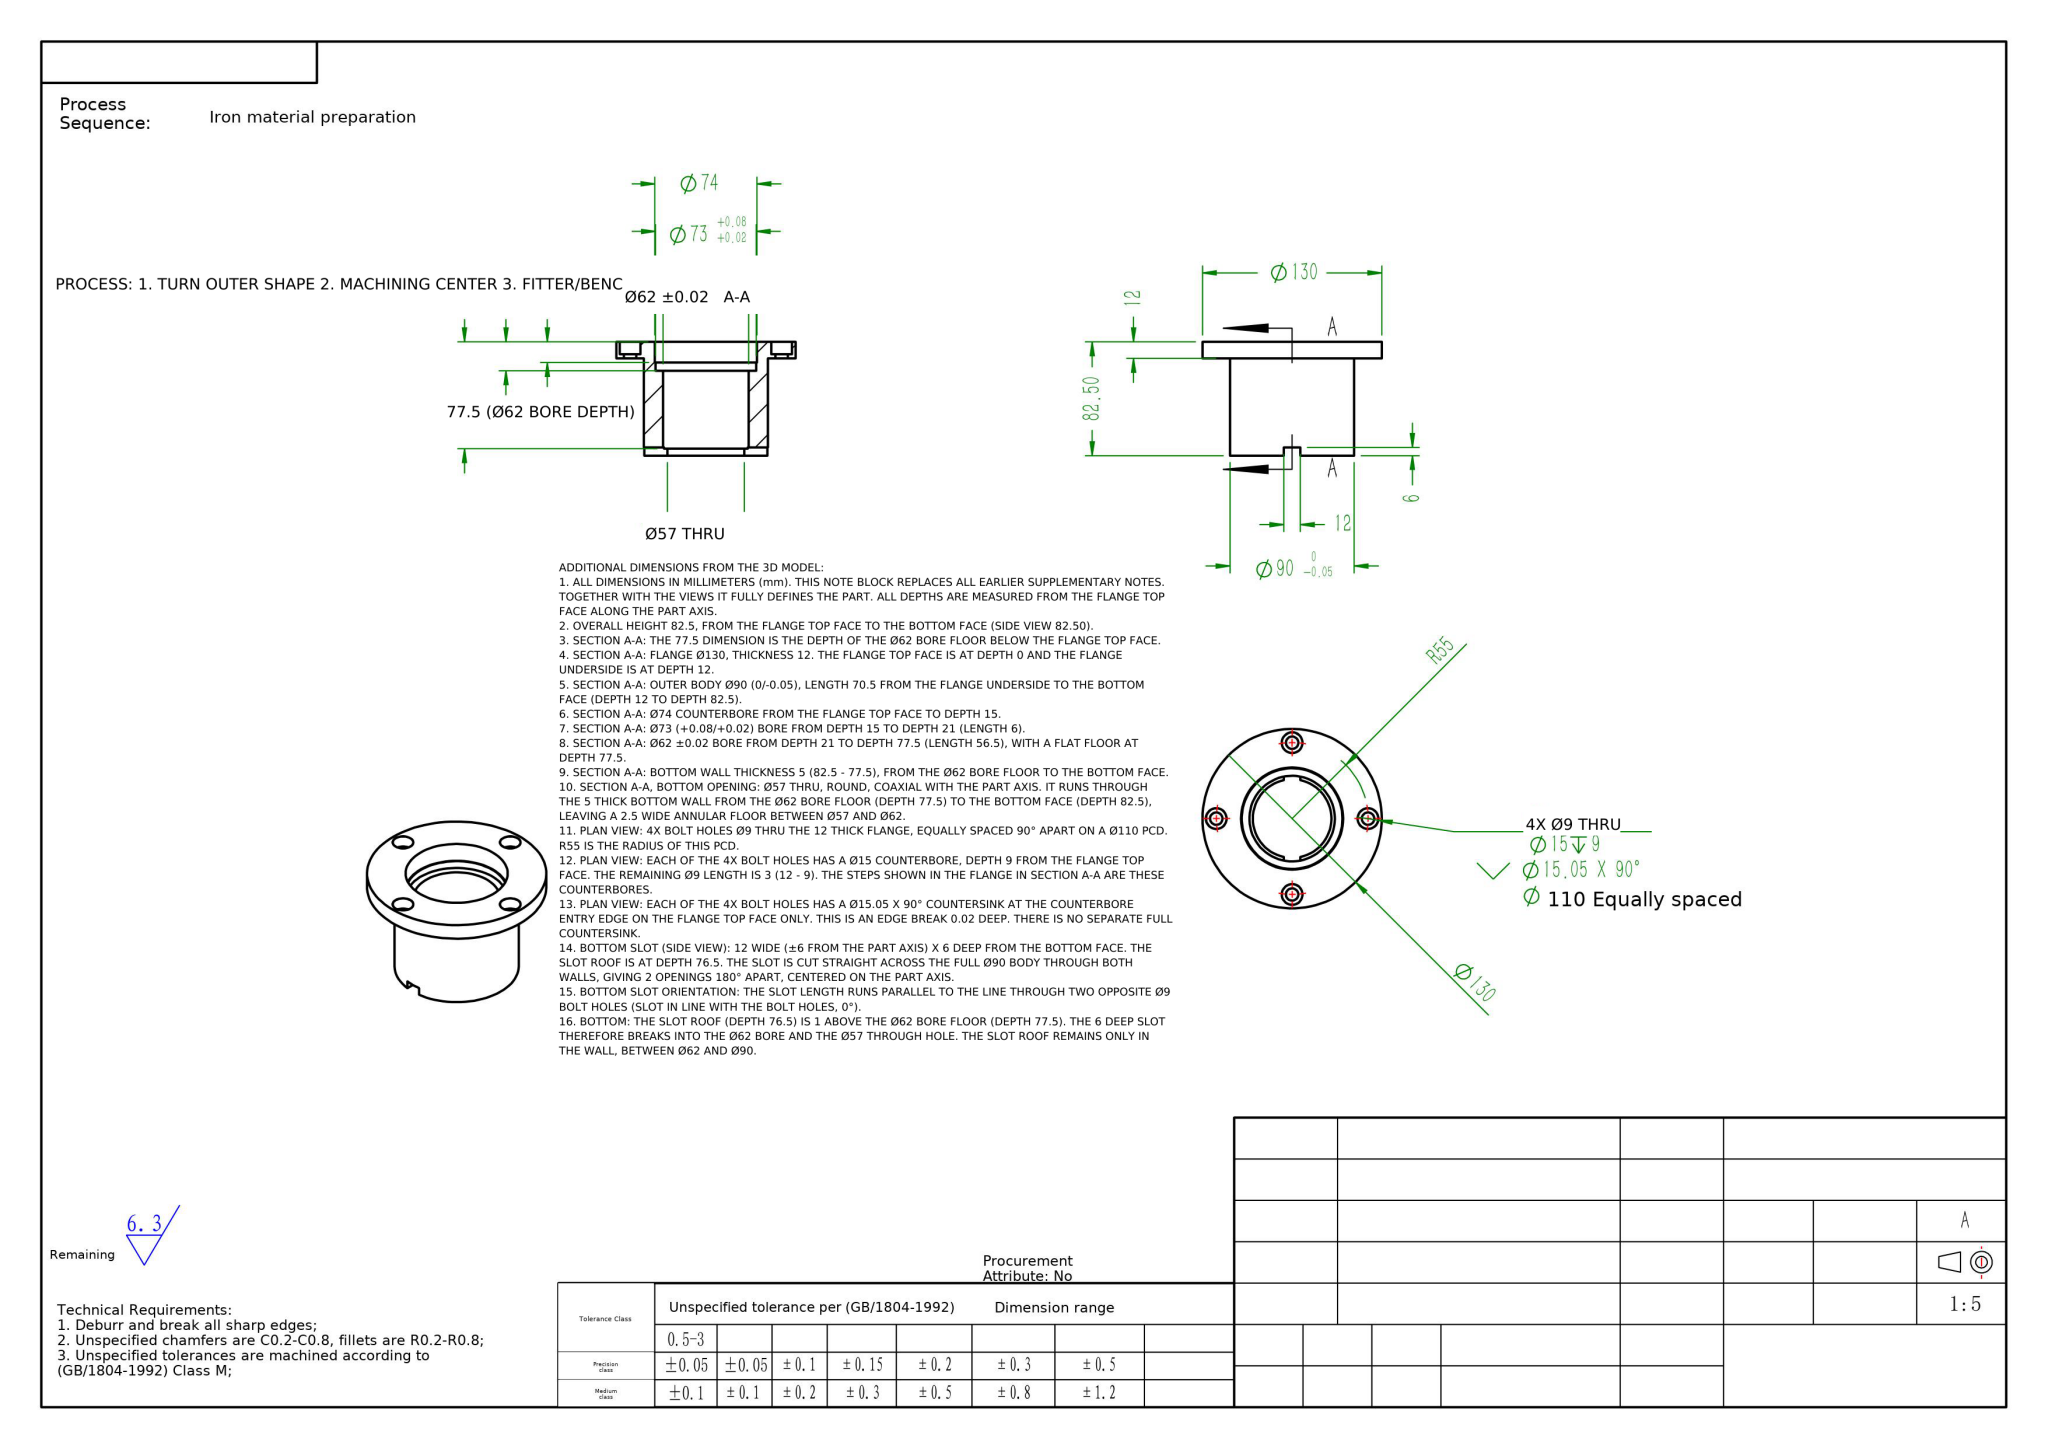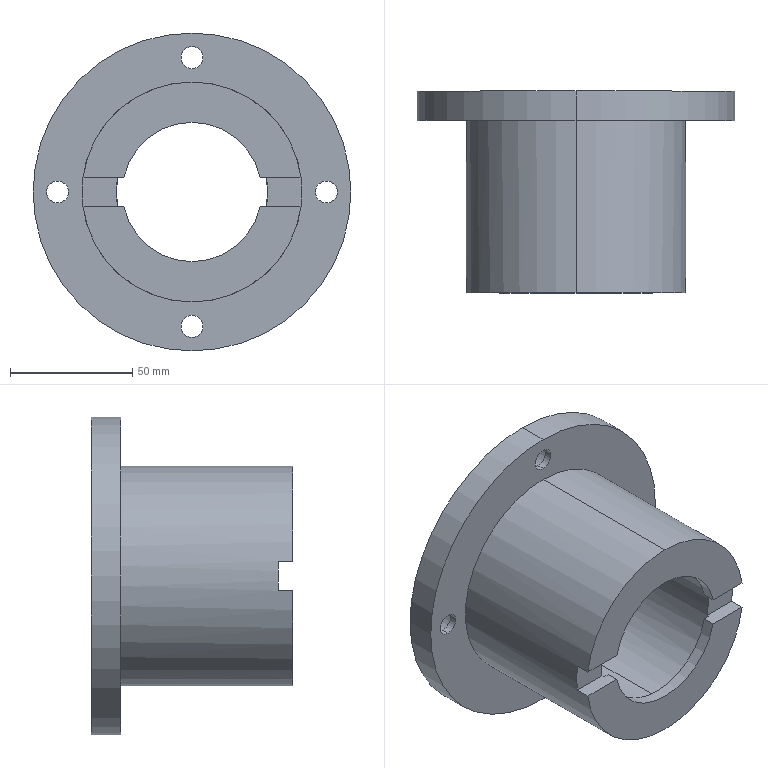Part | NX | mm | 1 solid | 55 faces | box 130 x 82.5 x 130 mm | volume 325367 mm3 | cylinder 29 | plane 18 | cone 8 | commonest cylinder face diameters 15 x8 9 x8 57 x3 130 x2 90 x2 62 x2 73 x2 74 x2